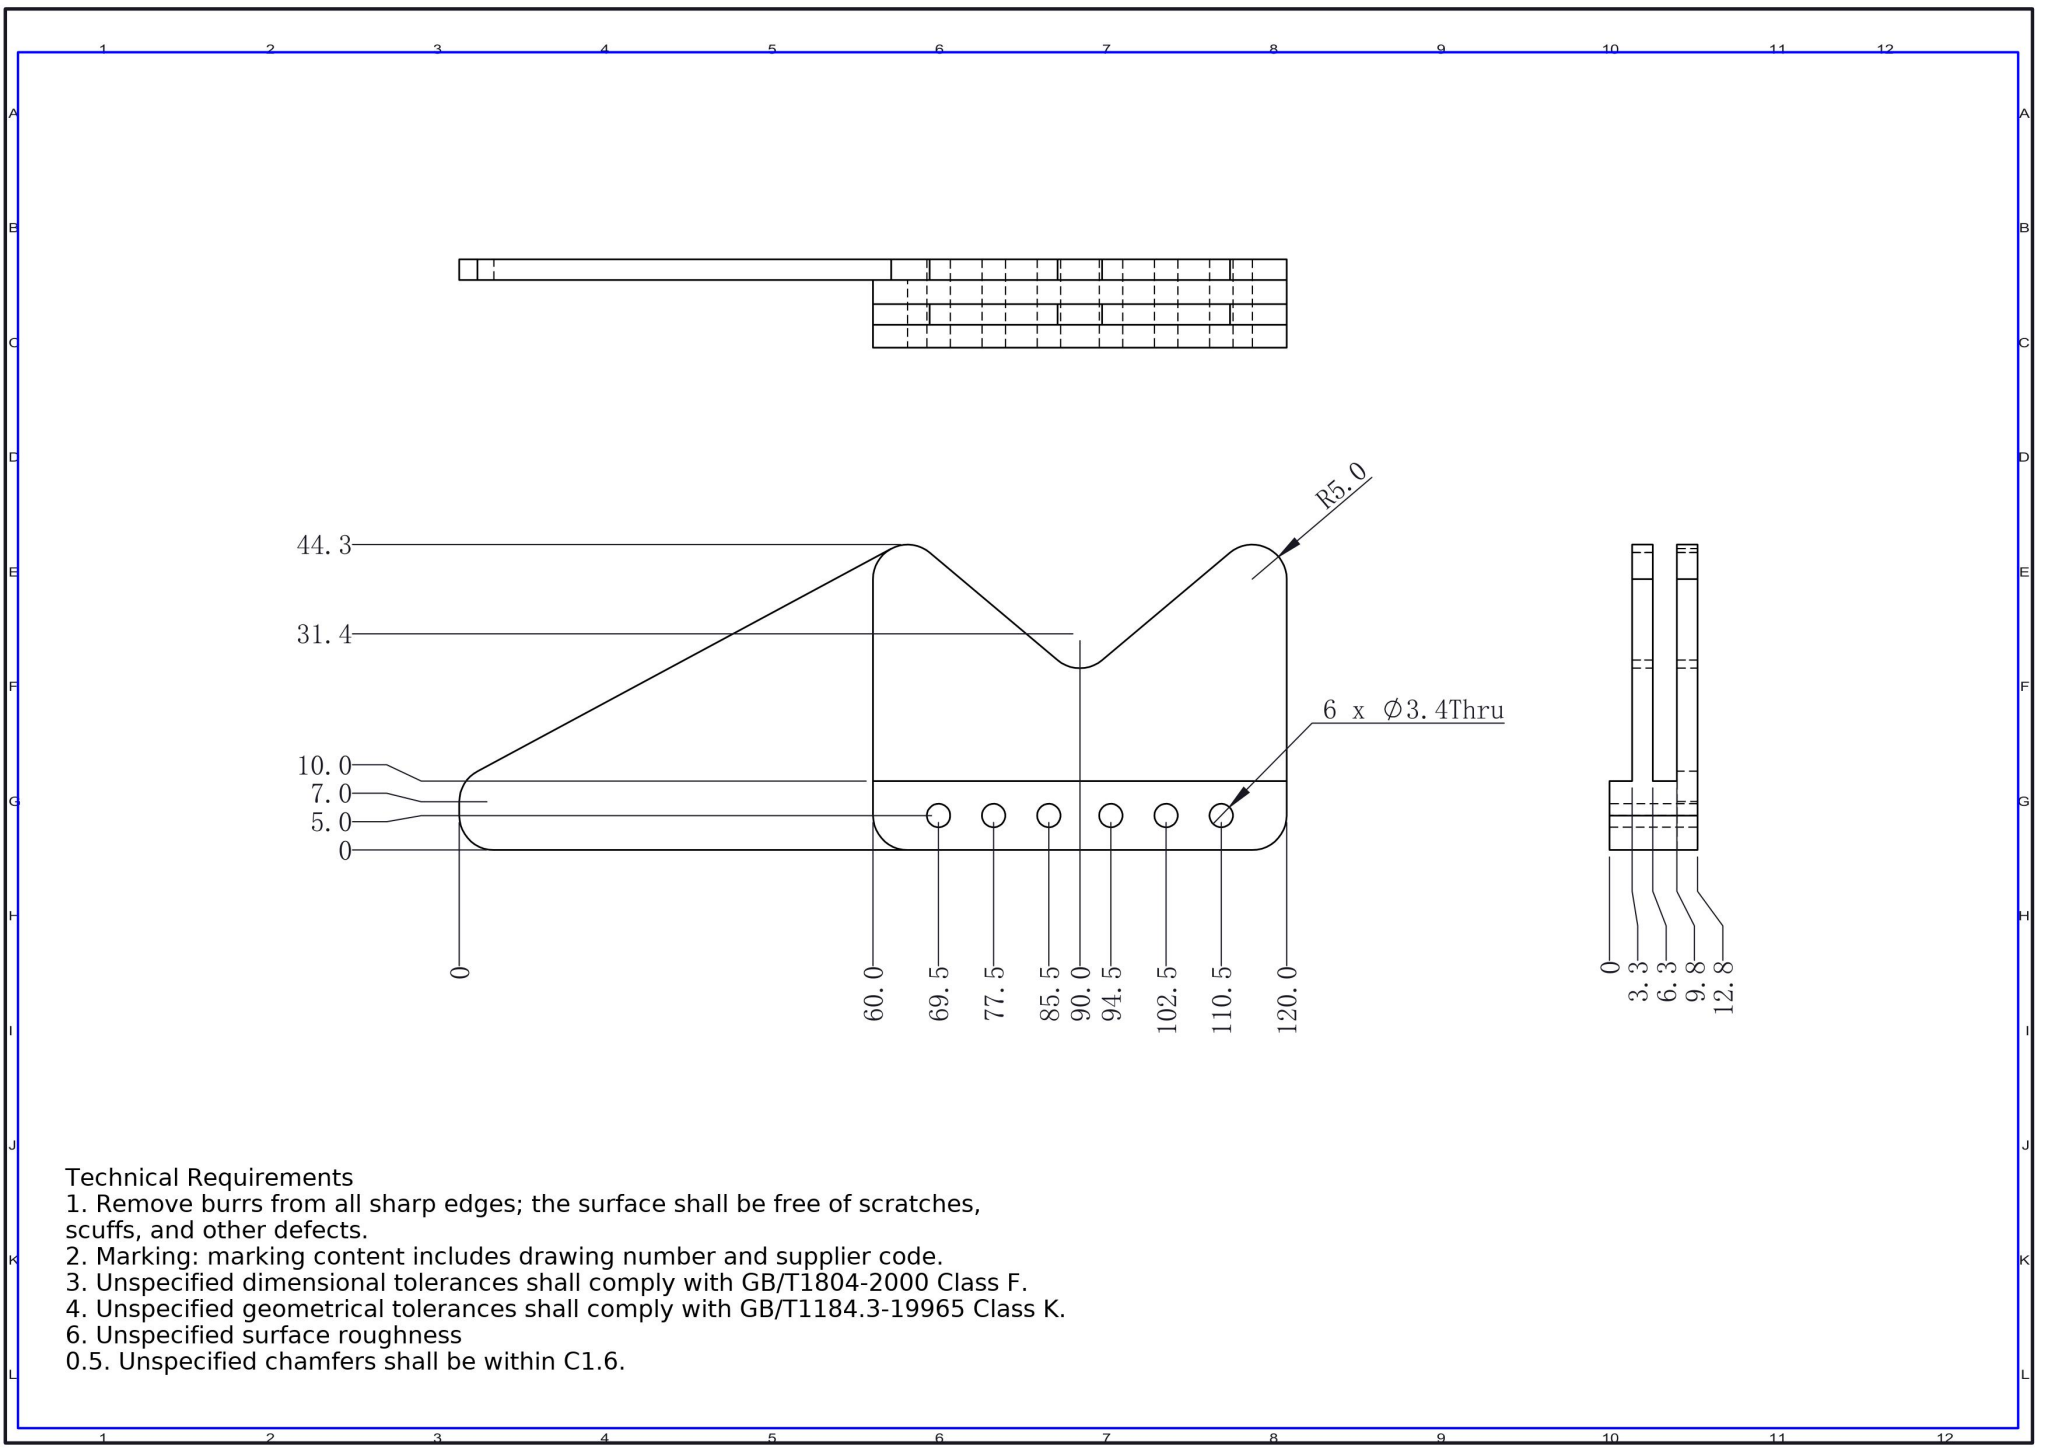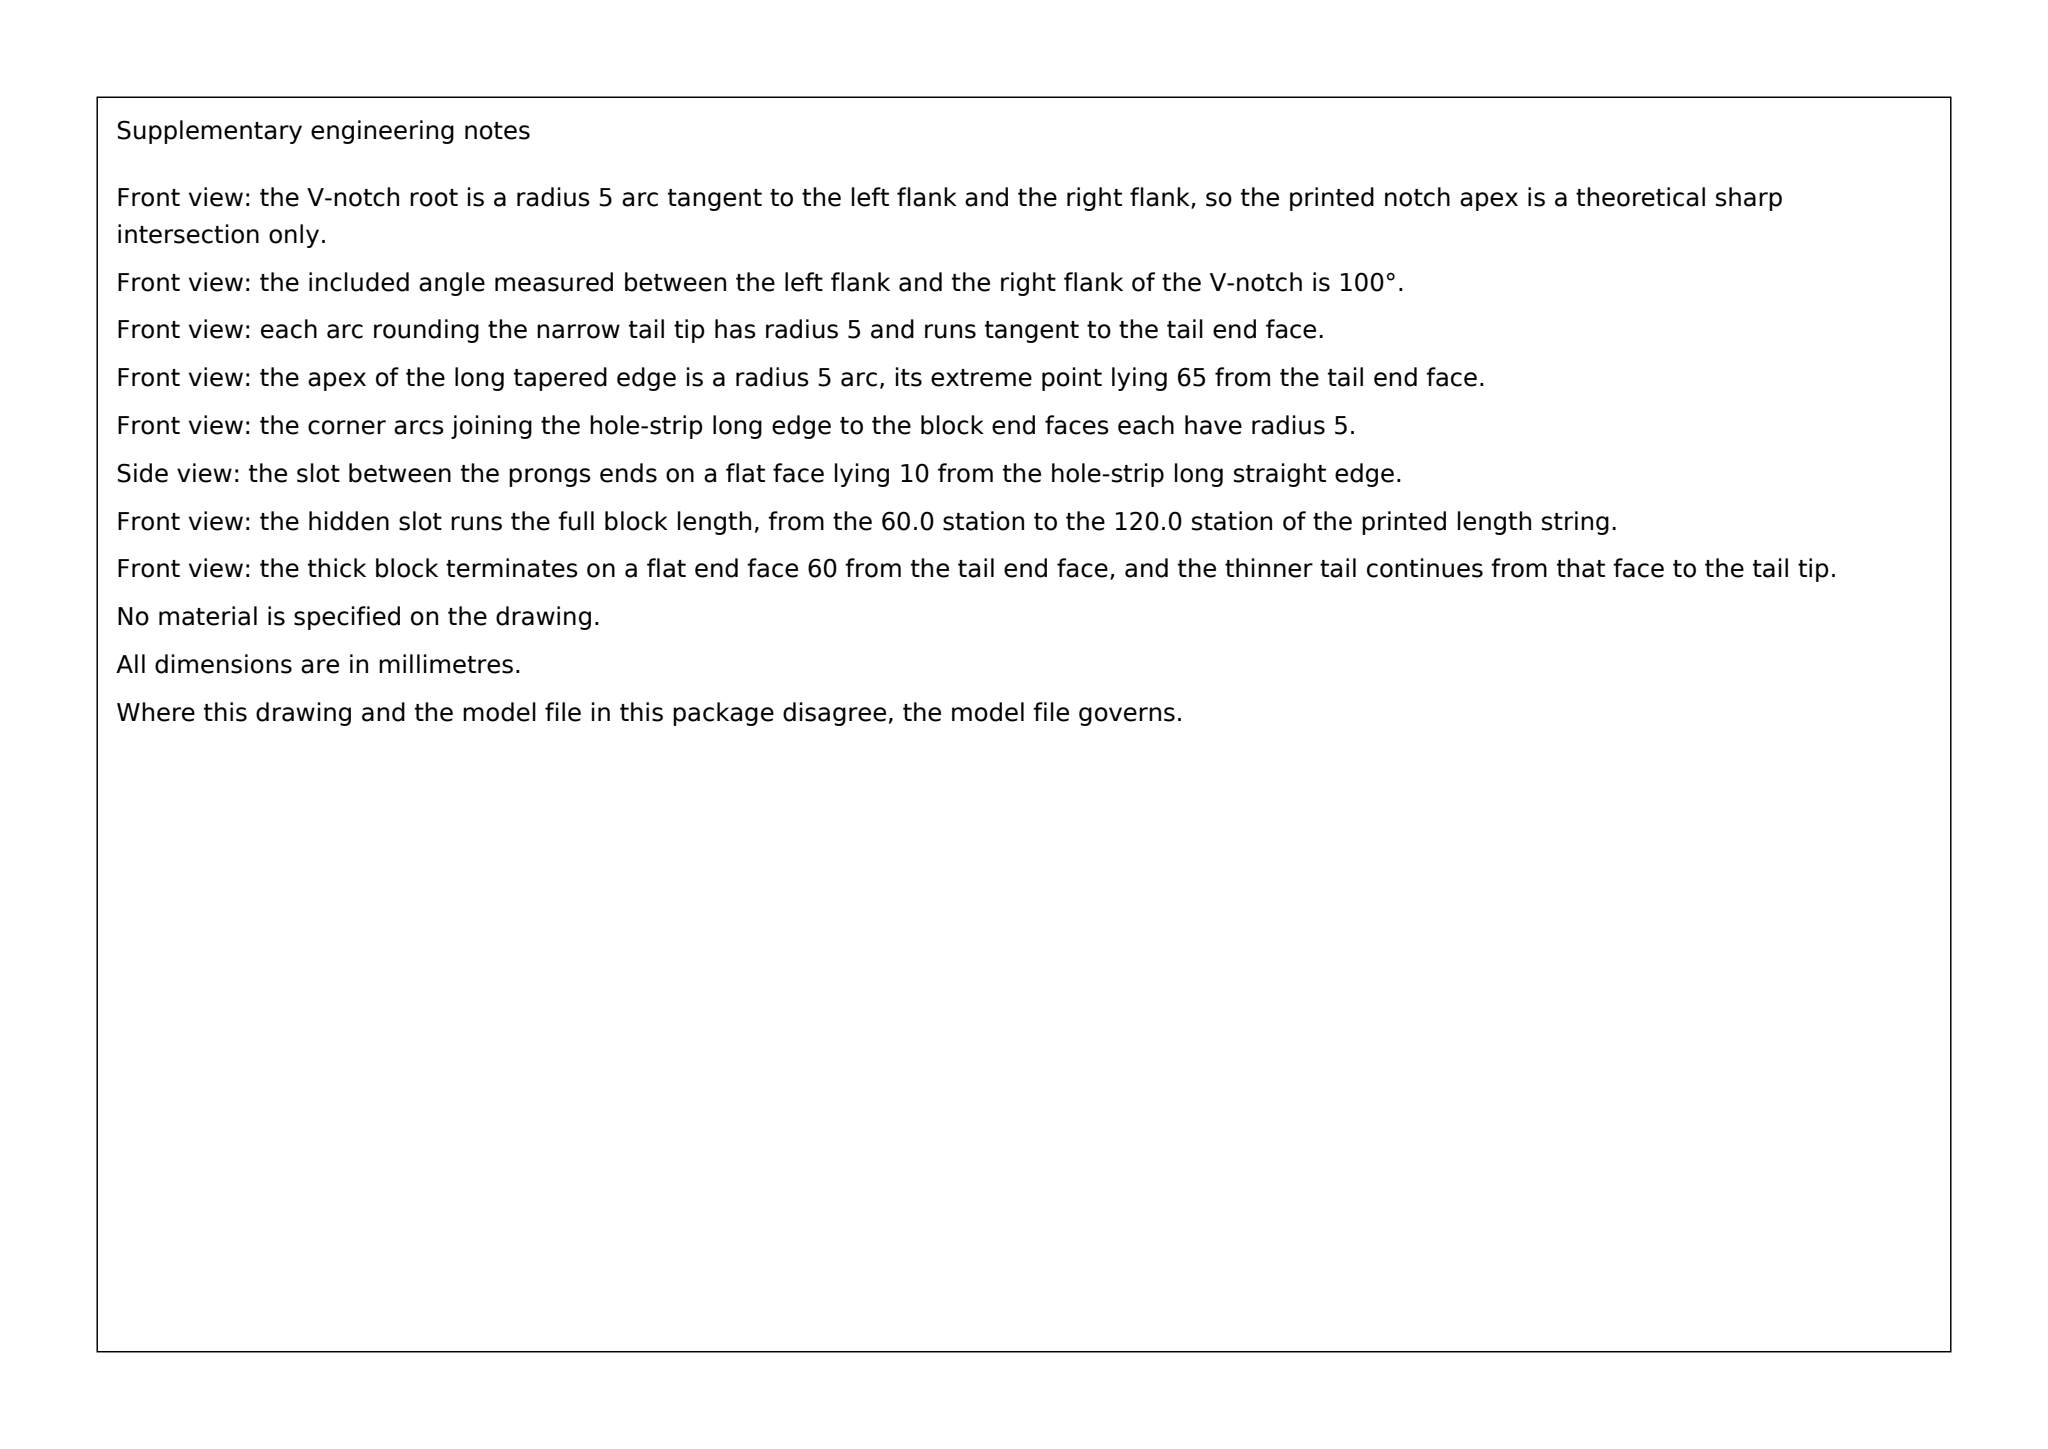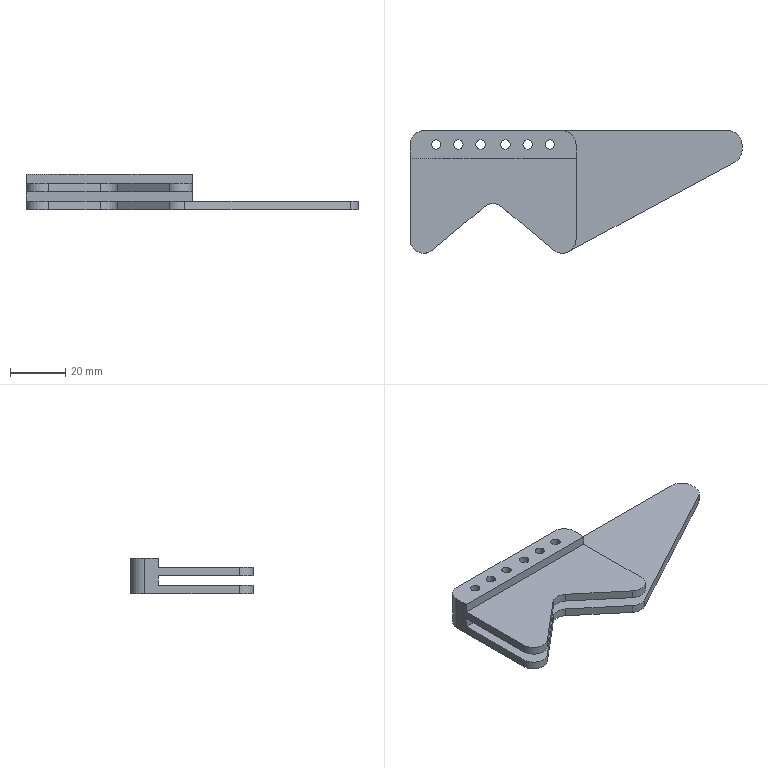Part | SolidWorks | mm | 1 solid | 38 faces | box 120 x 44.28 x 12.8 mm | volume 21136 mm3 | cylinder 22 | plane 16 | commonest cylinder face diameters 3.4 x12 10 x10
Drawing notes:
STEP THK: 3.0 THK X0-60, 12.8 THK X60-120 | from the solid: x planes 0/60/120; z planes 0/3.0/12.8; Ø10 fillets len 3.0 in thin zone, 12.8/9.8 in thick zone
6X Ø3.4 THRU, HOLE CL 5.0 FROM BTM EDGE (Y ORD 0) | from the solid: 6 cyl Ø3.4 axis z at y=39.28 of 44.277 bbox = 5.0 from datum edge; len 12.8 = THRU
LH DIAG EDGE 28.3° TO HORIZ, TAN R5 CL X5.0/Y7.0 TO R5 CL X65/Y39.3 | from the solid: Ø10 fillet cyls at STEP (115,37.27) & (55,5) -> dwg (5.0,7.01) & (65.0,39.28), both R5 len 3.0; external tangent line slope atan(32.27/60)=28.27°
TOP FLAT Y=44.28 RUNS X=65.0 TO X=115.0 (TAN PTS OF 2X R5) | from the solid: Y plane 44.28 (bbox y=44.277); R5 fillet CLs at dwg X=65.0 and X=115.0, Y=39.28 = 44.28-5 => tangent to top flat
TOP FLAT TO VALLEY EDGE 40° BELOW HORIZ; VALLEY R5 CL X90.0 Y31.36 | from the solid: Internal tangent between R5 CL (65.0,39.28) and valley R5 CL (90.0,31.36) [STEP (30,12.92)]: d=26.22, sin=10/26.22 -> 40.00°
VALLEY TO TOP-RH CORNER EDGE 40° UP FROM HORIZ; R5 CL X115.0 Y39.28 | from the solid: Internal tangent between valley R5 CL (90.0,31.36) and corner R5 CL (115.0,39.28) [STEP (5,5)]: d=26.22 -> 40.00°
TOP-RH APEX Y=44.28; EDGE X=120 TAN TO R5 AT Y=39.28 | from the solid: bbox y=44.277 top plane; x plane 0.0 (dwg X=120) right edge; R5 CL (115.0,39.28) tangent to both
SIDE VW Z STEPS 3.0/6.5/9.5 BREAK AT X=60.0; MAX THK 12.8 | from the solid: axis_planes x = 0.0, 60.0, 120.0 only; z planes 0, 3.0, 6.5, 9.5, 12.8; profile fillets len 3.0 (z0-3) vs R5 CL (65.0,5.0) len 9.8 (z3-12.8) tangent to X=60 face
SIDE VIEW Z ORDINATES: 0, 3.0, 6.5, 9.5, 12.8 (THK STEPS) | from the solid: axis_planes z = 0.0, 3.0, 6.5, 9.5, 12.8
3.0 THK WALLS: Z 0-3.0 FULL PROFILE; Z 6.5-9.5 X 60.0-120.0 | from the solid: z planes 0/3.0 and 6.5/9.5; R5 fillet faces count 2 at X>=60 (steps 55,5 / 30,12.92 / 5,5), count 1 at left end (115,37.27 / 115,39.28); x plane 60.0
SOLID BOSS 12.8 THK: X 60.0-120.0 x Y 0-10.0 FROM BTM EDGE | from the solid: x planes 60.0/120.0, y planes 34.28 (=Y10.0 from btm, 2 faces) & 44.28 (=Y0); R5 at X65,Y5 len 9.8 (Z3.0-12.8) and R5 at X115,Y5 len 12.8; 6x O3.4 thru 12.8 at Y5.0
OPEN GAPS Z 3.0-6.5 & Z 9.5-12.8 ABOVE Y 10.0, X 60.0-120.0 | from the solid: two coplanar faces at y=34.28 (Y10.0) bounding the Z3.0-6.5 and Z9.5-12.8 voids between the 3.0 walls
build123d program:
from build123d import *

# Parameters (mm, degrees)
SKETCH1_W            = 60
SKETCH1_H            = 50
BOSS_EXTRUDE1_DEPTH  = 9.8
SKETCH2_W            = 60
SKETCH2_H            = 3.5
SKETCH2_H_2          = 3.3
CUT_EXTRUDE1_DEPTH   = 40
CUT_EXTRUDE2_DEPTH   = 15
FILLET1_R            = 5
BOSS_EXTRUDE2_DEPTH  = 3
M3_CLEARANCE_HOLE1_D = 3.4
FILLET2_R            = 5
FILLET3_R            = 5
FILLET5_R            = 5


with BuildPart() as part:
    # Sketch1 → Boss-Extrude1 (new body)
    with BuildSketch(Plane.XY):
        Rectangle(SKETCH1_W, SKETCH1_H)
    extrude(amount=BOSS_EXTRUDE1_DEPTH)

    # Sketch2 → Cut-Extrude1 (cut)
    with BuildSketch(Plane.XZ.offset(25)):
        with Locations((0, 1.75)):
            Rectangle(SKETCH2_W, SKETCH2_H)
        with Locations((0, 8.15)):
            Rectangle(SKETCH2_W, SKETCH2_H_2)
    extrude(amount=-CUT_EXTRUDE1_DEPTH, mode=Mode.SUBTRACT)

    # Sketch3 → Cut-Extrude2 (cut)
    with BuildSketch(Plane.XY.offset(9.8)):
        Polygon((-30, -25), (0, 0.173), (30, -25), align=None)
    extrude(amount=-CUT_EXTRUDE2_DEPTH, mode=Mode.SUBTRACT)

    # Fillet1
    fillet1_edges = [part.edges().sort_by_distance(p)[0] for p in [
        (30, -25, 5),
        (-30, -25, 5),
    ]]
    fillet(fillet1_edges, radius=FILLET1_R)

    # Sketch9 → Boss-Extrude2 (add)
    with BuildSketch(Plane(origin=(0, 0, 0), x_dir=(-1, 0, 0), z_dir=(0, 0, -1))):
        Polygon((30, 25), (30, -25), (0, 0.173), (-24.383, -20.287), (-90, 15), (-90, 25), align=None)
    extrude(amount=BOSS_EXTRUDE2_DEPTH)

    # M3 Clearance Hole1 (through all)
    with Locations(Plane.XY.offset(9.8)):
        with Locations((-12.5, 20), (12.5, 20), (-20.5, 20), (-4.5, 20), (4.5, 20), (20.5, 20)):
            Hole(M3_CLEARANCE_HOLE1_D / 2)

    # Fillet2
    fillet2_edges = [part.edges().sort_by_distance(p)[0] for p in [
        (-30, 25, 3.4),
        (30, 25, 4.9),
    ]]
    fillet(fillet2_edges, radius=FILLET2_R)

    # Fillet3
    fillet3_edges = [part.edges().sort_by_distance(p)[0] for p in [
        (0, 0.173, 5),
        (0, 0.173, -1.5),
    ]]
    fillet(fillet3_edges, radius=FILLET3_R)

    # Fillet5
    fillet5_edges = [part.edges().sort_by_distance(p)[0] for p in [
        (90, 25, -1.5),
        (90, 15, -1.5),
        (24.383, -20.287, -1.5),
        (-30, -25, -1.5),
    ]]
    fillet(fillet5_edges, radius=FILLET5_R)


solid = part.part